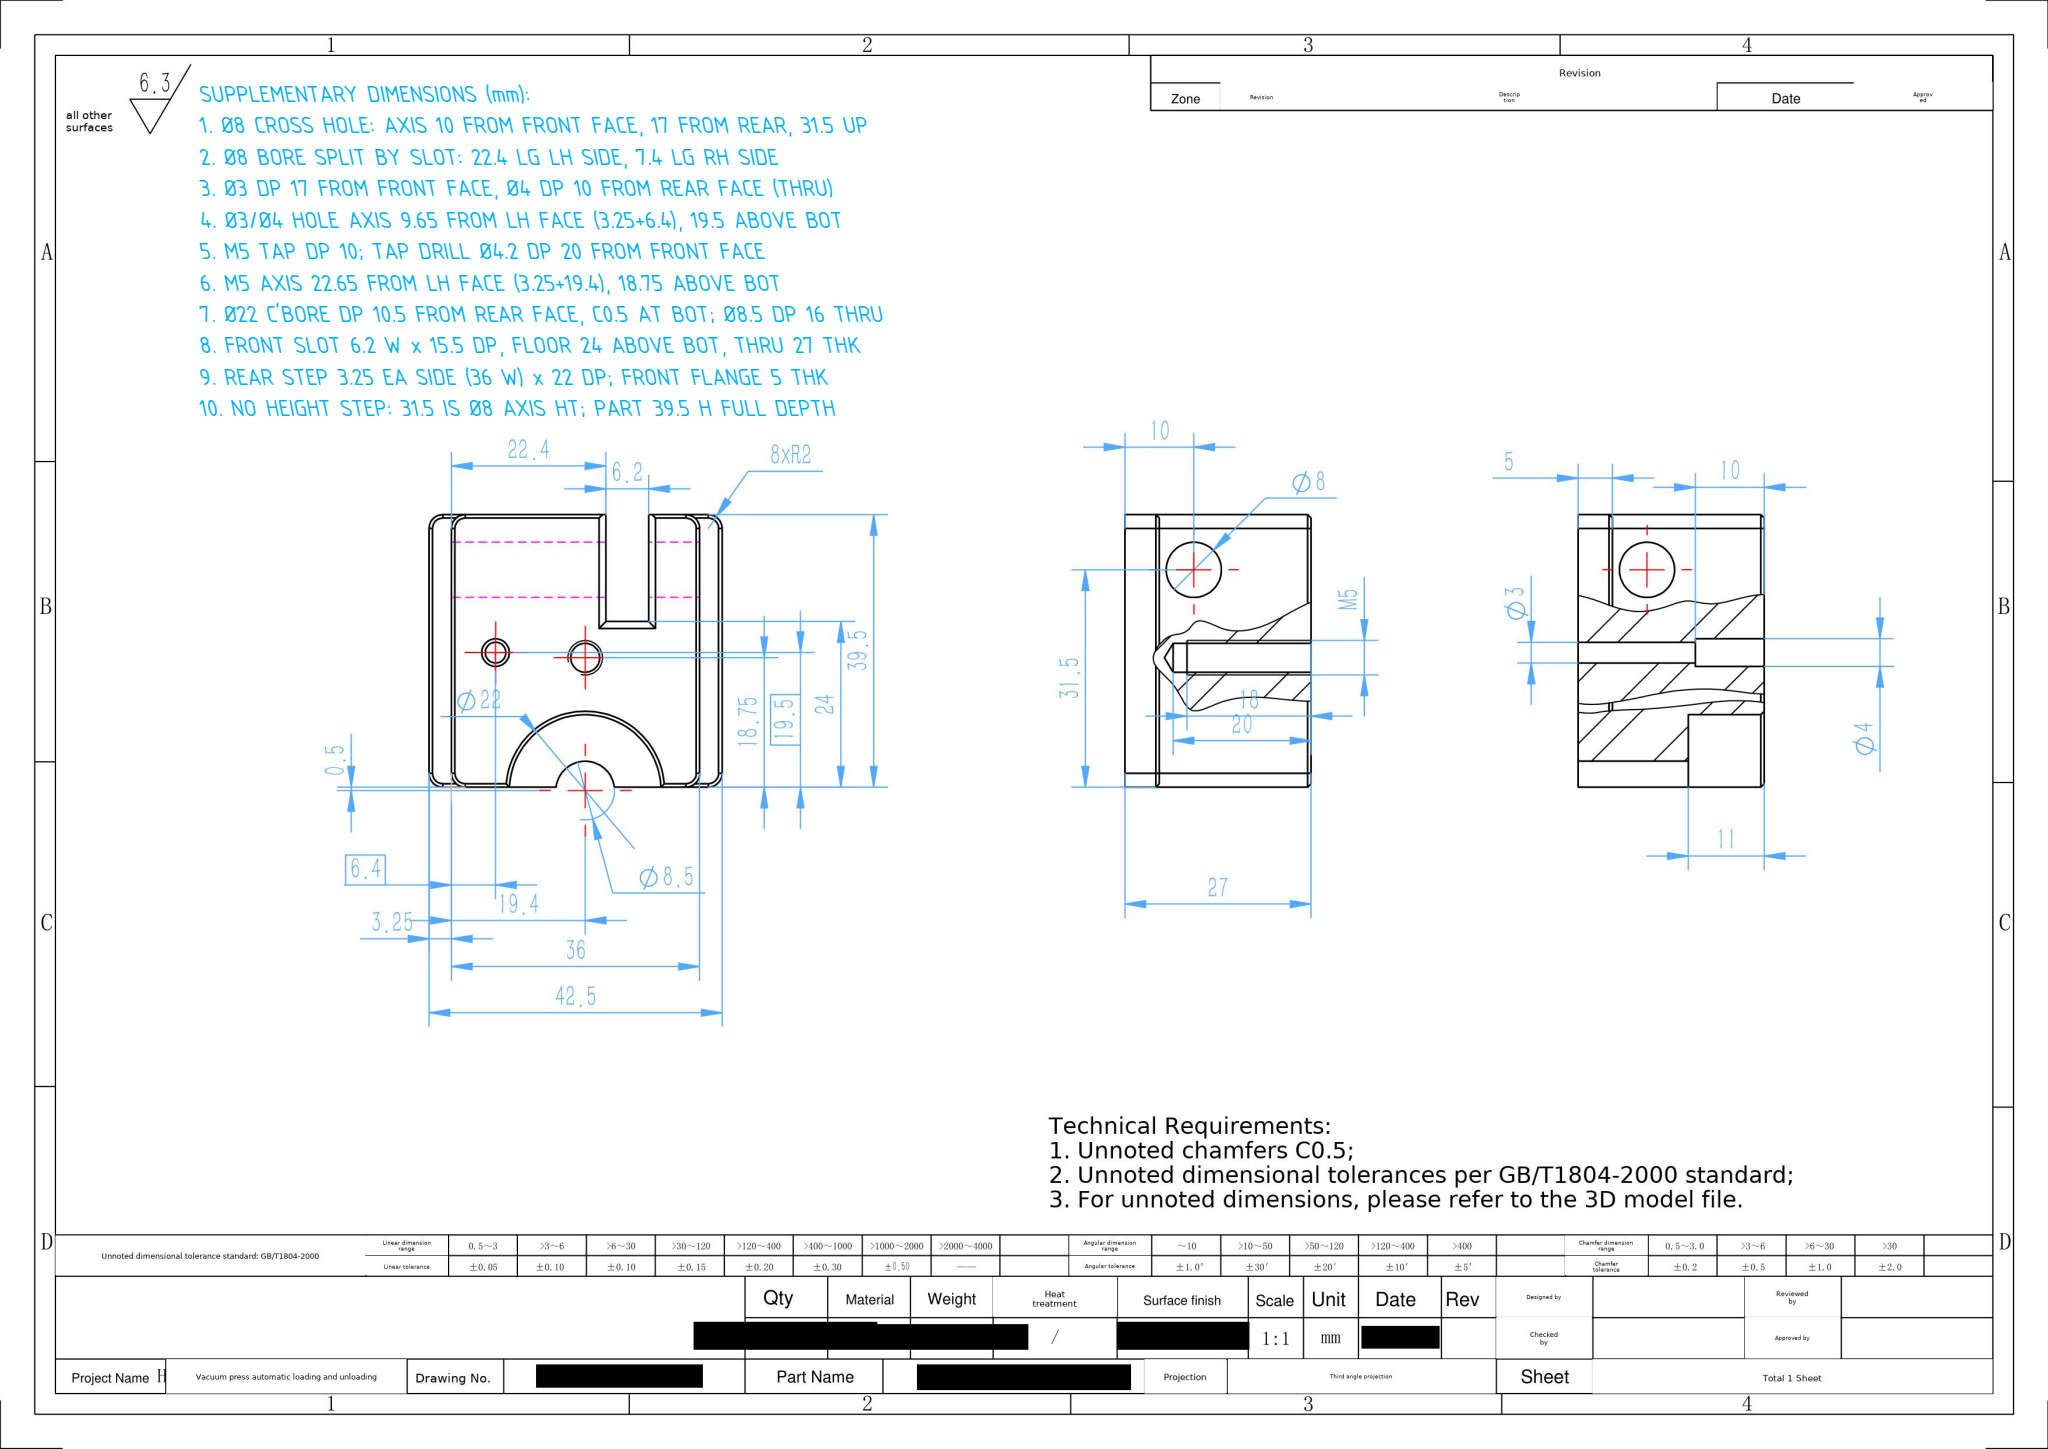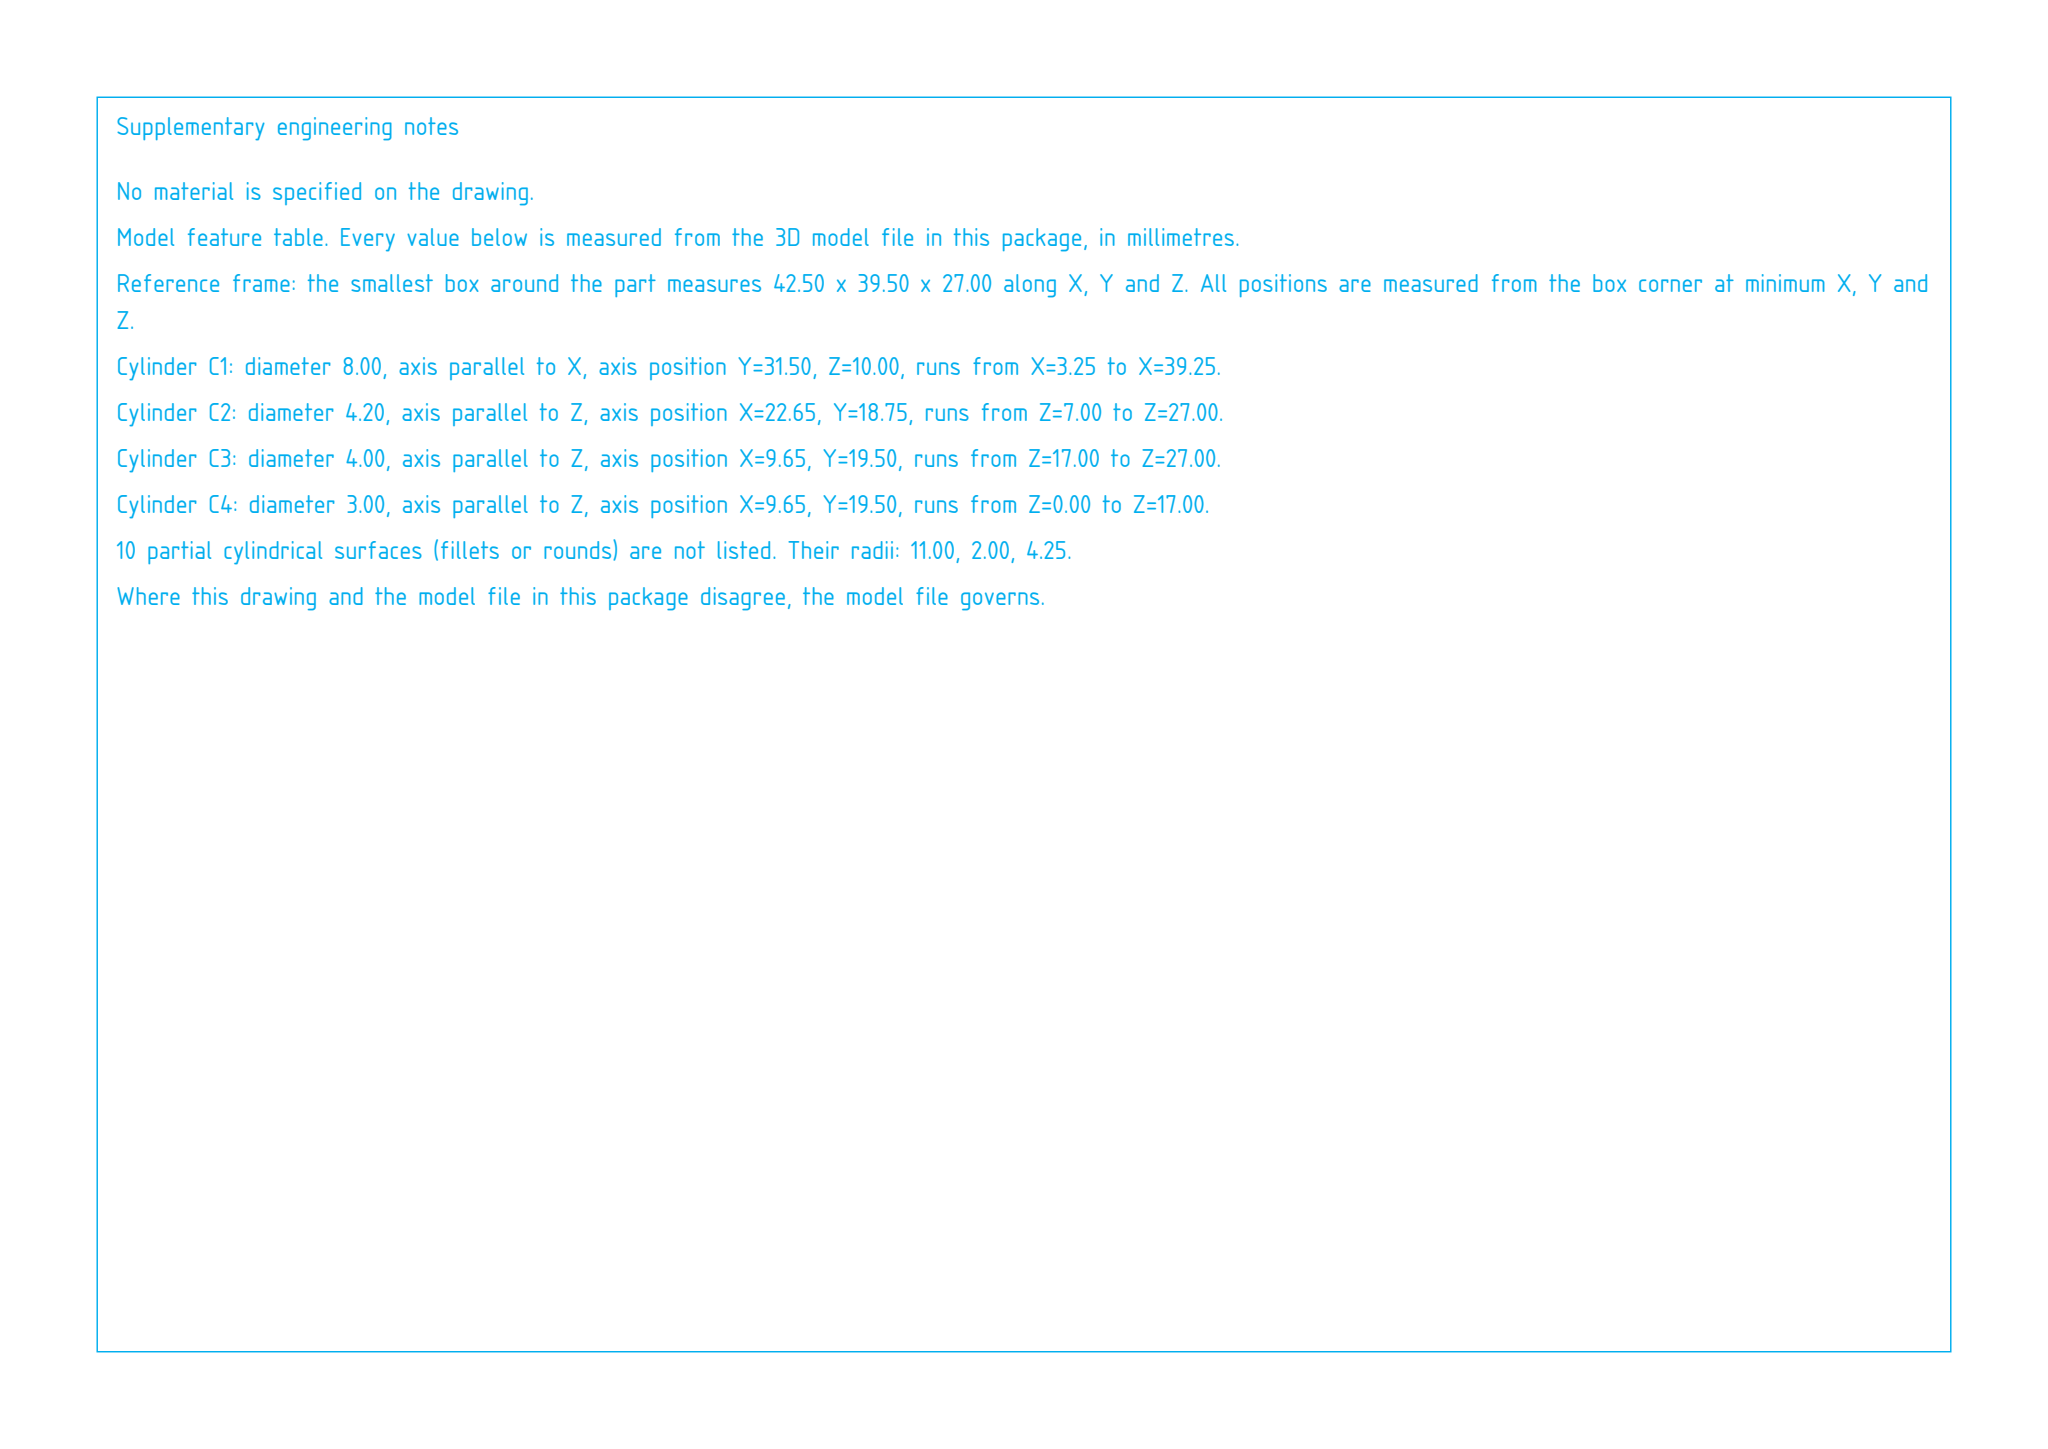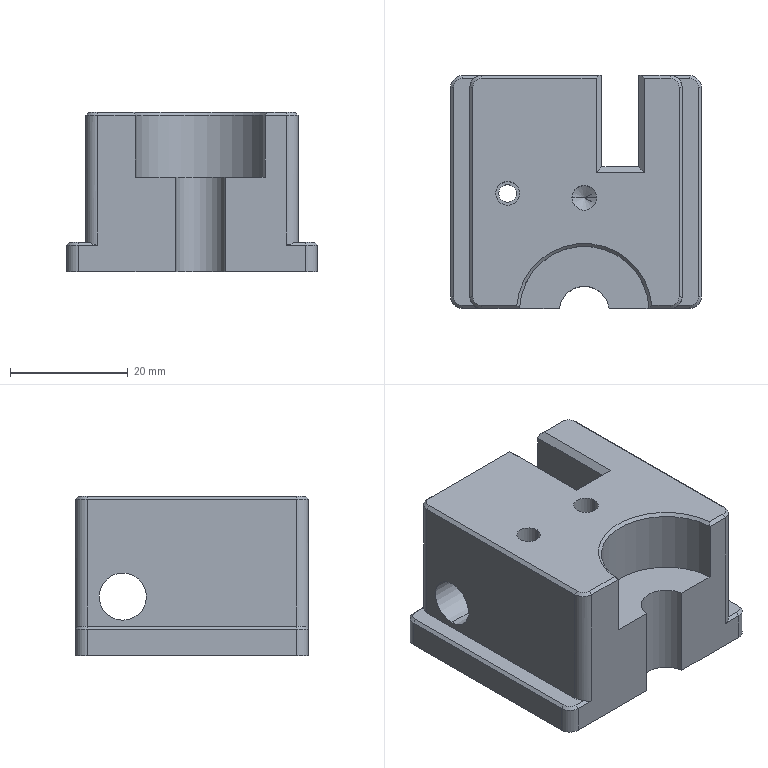Part | SolidWorks | mm | 1 solid | 63 faces | box 42.5 x 39.5 x 27 mm | volume 32558 mm3 | plane 32 | cylinder 20 | cone 11 | commonest cylinder face diameters 4 x10 8 x4 4.2 x2 3 x2 8.5 x1 22 x1
build123d program:
from build123d import *

# Parameters (mm, degrees)
SKETCH1_W             = 42.5
SKETCH1_H             = 39.5
BOSS_EXTRUDE1_DEPTH   = 5
SKETCH2_W             = 36
SKETCH2_H             = 39.5
BOSS_EXTRUDE2_DEPTH   = 22
FILLET1_R             = 2
SKETCH3_R             = 4.25
CUT_EXTRUDE1_DEPTH    = 40.631
SKETCH4_R             = 11
CUT_EXTRUDE2_DEPTH    = 11
SKETCH5_R             = 4
CUT_EXTRUDE3_DEPTH    = 52.572
SKETCH6_W             = 6.2
SKETCH6_H             = 15.5
CUT_EXTRUDE4_DEPTH    = 40.631
M5_TAPPED_HOLE1_D     = 4.2
M5_TAPPED_HOLE1_DEPTH = 20
M5_TAPPED_HOLE1_TIP   = 1.262
SKETCH9_R             = 1.5
CUT_EXTRUDE5_DEPTH    = 40.631
SKETCH10_R            = 2
CUT_EXTRUDE6_DEPTH    = 10
CHAMFER1_SIZE         = 1
CHAMFER2_SIZE         = 0.5


with BuildPart() as part:
    # Sketch1 → Boss-Extrude1 (new body)
    with BuildSketch(Plane.XY):
        Rectangle(SKETCH1_W, SKETCH1_H)
    extrude(amount=BOSS_EXTRUDE1_DEPTH)

    # Sketch2 → Boss-Extrude2 (add)
    with BuildSketch(Plane.XY.offset(5)):
        Rectangle(SKETCH2_W, SKETCH2_H)
    extrude(amount=BOSS_EXTRUDE2_DEPTH)

    # Fillet1
    fillet1_edges = [part.edges().sort_by_distance(p)[0] for p in [
        (18, -19.75, 16),
        (18, 19.75, 16),
        (-18, 19.75, 16),
        (-18, -19.75, 16),
        (21.25, -19.75, 2.5),
        (-21.25, -19.75, 2.5),
        (-21.25, 19.75, 2.5),
        (21.25, 19.75, 2.5),
    ]]
    fillet(fillet1_edges, radius=FILLET1_R)

    # Sketch3 → Cut-Extrude1 (cut, through all)
    with BuildSketch(Plane.XY.offset(27)):
        with Locations((1.4, -20.25)):
            Circle(SKETCH3_R)
    extrude(amount=-CUT_EXTRUDE1_DEPTH, mode=Mode.SUBTRACT)

    # Sketch4 → Cut-Extrude2 (cut)
    with BuildSketch(Plane.XY.offset(27)):
        with Locations((1.4, -20.25)):
            Circle(SKETCH4_R)
    extrude(amount=-CUT_EXTRUDE2_DEPTH, mode=Mode.SUBTRACT)

    # Sketch5 → Cut-Extrude3 (cut, through all)
    with BuildSketch(Plane.ZY.offset(18)):
        with Locations((10, 11.75)):
            Circle(SKETCH5_R)
    extrude(amount=-CUT_EXTRUDE3_DEPTH, mode=Mode.SUBTRACT)

    # Sketch6 → Cut-Extrude4 (cut, through all)
    with BuildSketch(Plane.XY.offset(27)):
        with Locations((7.5, 12)):
            Rectangle(SKETCH6_W, SKETCH6_H)
    extrude(amount=-CUT_EXTRUDE4_DEPTH, mode=Mode.SUBTRACT)

    # M5 Tapped Hole1
    with Locations(Plane.XY.offset(27)):
        with Locations((1.4, -1)):
            Hole(M5_TAPPED_HOLE1_D / 2, depth=M5_TAPPED_HOLE1_DEPTH)
            with Locations((0, 0, -(M5_TAPPED_HOLE1_DEPTH + M5_TAPPED_HOLE1_TIP / 2))):  # 118° drill point
                Cone(0, M5_TAPPED_HOLE1_D / 2, M5_TAPPED_HOLE1_TIP, mode=Mode.SUBTRACT)

    # Sketch9 → Cut-Extrude5 (cut, through all)
    with BuildSketch(Plane.XY.offset(27)):
        with Locations((-11.6, -0.25)):
            Circle(SKETCH9_R)
    extrude(amount=-CUT_EXTRUDE5_DEPTH, mode=Mode.SUBTRACT)

    # Sketch10 → Cut-Extrude6 (cut)
    with BuildSketch(Plane.XY.offset(27)):
        with Locations((-11.6, -0.25)):
            Circle(SKETCH10_R)
    extrude(amount=-CUT_EXTRUDE6_DEPTH, mode=Mode.SUBTRACT)

    # Chamfer1
    chamfer1_edges = [part.edges().sort_by_distance(p)[0] for p in [
        (4.4, 12, 27),
        (7.5, 4.25, 27),
        (10.6, 12, 27),
    ]]
    chamfer(chamfer1_edges, length=CHAMFER1_SIZE)

    # Chamfer2
    chamfer2_edges = [part.edges().sort_by_distance(p)[0] for p in [
        (-17.625, 19.75, 5),
        (-20.664, 19.164, 5),
        (-21.25, 0, 5),
        (17.625, -19.75, 5),
        (-20.664, -19.164, 5),
        (17.625, 19.75, 5),
        (20.664, 19.164, 5),
        (21.25, 0, 5),
        (20.664, -19.164, 5),
        (13.8, 19.75, 27),
        (17.414, 19.164, 27),
        (-6.3, 19.75, 27),
        (-17.414, 19.164, 27),
        (-18, 0, 27),
        (-17.414, -19.164, 27),
        (-12.794, -19.75, 27),
        (1.4, -9.25, 27),
        (17.414, -19.164, 27),
        (18, 0, 27),
    ]]
    chamfer(chamfer2_edges, length=CHAMFER2_SIZE)


solid = part.part